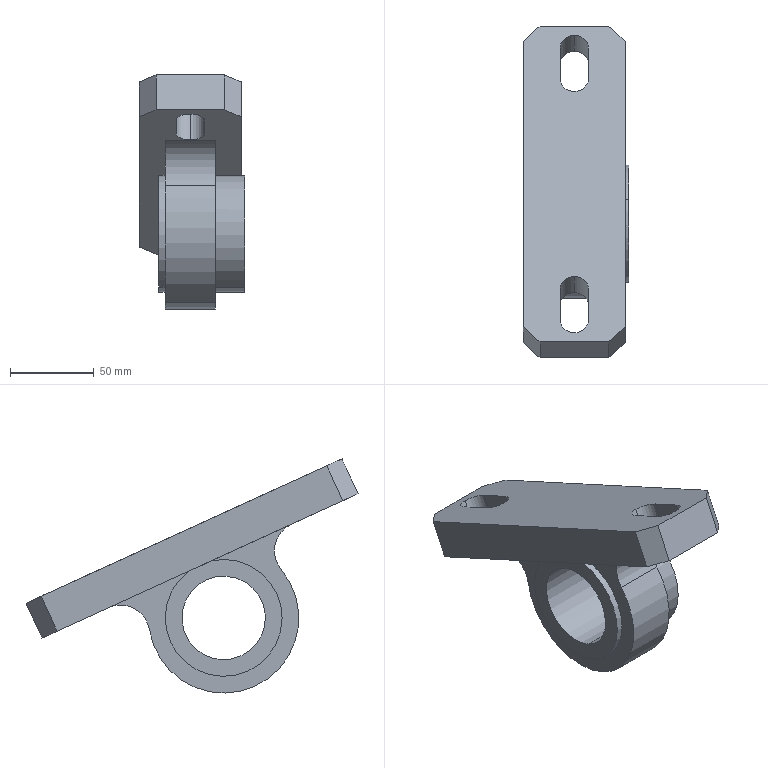Component | SolidWorks | Z90510-1 | 1 solid | 34 faces | box 63.1 x 198.79 x 140.2 mm | volume 431152 mm3 | plane 18 | cylinder 16 | commonest cylinder face diameters 17 x6 70 x4 90 x2 50 x2 35 x2
STEP:
#1=COLOUR_RGB('',0.7922,0.8196,0.9333);
#2=FILL_AREA_STYLE_COLOUR('',#1);
#3=FILL_AREA_STYLE('',(#2));
#4=SURFACE_STYLE_FILL_AREA(#3);
#5=SURFACE_SIDE_STYLE('',(#4));
#6=SURFACE_STYLE_USAGE(.BOTH.,#5);
#7=PRESENTATION_STYLE_ASSIGNMENT((#6));
#8=CARTESIAN_POINT('',(27.492,0.6244,-1.612));
#9=VERTEX_POINT('',#8);
#10=CARTESIAN_POINT('',(27.492,3.109,-0.2777));
#11=VERTEX_POINT('',#10);
#12=CARTESIAN_POINT('',(27.492,1.36,0.));
#13=DIRECTION('',(1.,0.,0.));
#14=DIRECTION('',(0.,0.4149,0.9099));
#15=AXIS2_PLACEMENT_3D('',#12,#13,#14);
#16=CIRCLE('',#15,1.772);
#17=EDGE_CURVE('',#9,#11,#16,.T.);
#18=ORIENTED_EDGE('',*,*,#17,.F.);
#19=CARTESIAN_POINT('',(26.311,0.6244,-1.612));
#20=VERTEX_POINT('',#19);
#21=CARTESIAN_POINT('',(27.374,0.6244,-1.612));
#22=DIRECTION('',(-1.,0.,0.));
#23=VECTOR('',#22,39.37);
#24=LINE('',#21,#23);
#25=EDGE_CURVE('',#9,#20,#24,.T.);
#26=ORIENTED_EDGE('',*,*,#25,.T.);
#27=CARTESIAN_POINT('',(26.311,3.109,-0.2777));
#28=VERTEX_POINT('',#27);
#29=CARTESIAN_POINT('',(26.311,1.36,0.));
#30=DIRECTION('',(1.,0.,0.));
#31=DIRECTION('',(0.,0.4149,0.9099));
#32=AXIS2_PLACEMENT_3D('',#29,#30,#31);
#33=CIRCLE('',#32,1.772);
#34=EDGE_CURVE('',#20,#28,#33,.T.);
#35=ORIENTED_EDGE('',*,*,#34,.T.);
#36=CARTESIAN_POINT('',(27.492,3.109,-0.2777));
#37=DIRECTION('',(-1.,0.,0.));
#38=VECTOR('',#37,39.37);
#39=LINE('',#36,#38);
#40=EDGE_CURVE('',#11,#28,#39,.T.);
#41=ORIENTED_EDGE('',*,*,#40,.F.);
#42=EDGE_LOOP('',(#18,#26,#35,#41));
#43=FACE_OUTER_BOUND('',#42,.T.);
#44=CARTESIAN_POINT('',(27.374,1.36,0.));
#45=DIRECTION('',(-1.,0.,0.));
#46=DIRECTION('',(0.,-0.4149,-0.9099));
#47=AXIS2_PLACEMENT_3D('',#44,#45,#46);
#48=CYLINDRICAL_SURFACE('',#47,1.772);
#49=ADVANCED_FACE('',(#43),#48,.T.);
#50=CARTESIAN_POINT('',(26.902,5.804,0.4481));
#51=VERTEX_POINT('',#50);
#52=CARTESIAN_POINT('',(27.236,5.5,0.587));
#53=VERTEX_POINT('',#52);
#54=CARTESIAN_POINT('',(26.902,5.5,0.587));
#55=DIRECTION('',(0.,-0.4149,-0.9099));
#56=DIRECTION('',(0.,-0.9099,0.4149));
#57=AXIS2_PLACEMENT_3D('',#54,#55,#56);
#58=CIRCLE('',#57,0.3346);
#59=EDGE_CURVE('',#51,#53,#58,.T.);
#60=ORIENTED_EDGE('',*,*,#59,.F.);
#61=CARTESIAN_POINT('',(26.902,5.429,-0.3758));
#62=VERTEX_POINT('',#61);
#63=CARTESIAN_POINT('',(26.902,5.804,0.4481));
#64=DIRECTION('',(0.,-0.4149,-0.9099));
#65=VECTOR('',#64,39.37);
#66=LINE('',#63,#65);
#67=EDGE_CURVE('',#51,#62,#66,.T.);
#68=ORIENTED_EDGE('',*,*,#67,.T.);
#69=CARTESIAN_POINT('',(27.236,5.124,-0.2369));
#70=VERTEX_POINT('',#69);
#71=CARTESIAN_POINT('',(26.902,5.124,-0.2369));
#72=DIRECTION('',(0.,-0.4149,-0.9099));
#73=DIRECTION('',(0.,-0.9099,0.4149));
#74=AXIS2_PLACEMENT_3D('',#71,#72,#73);
#75=CIRCLE('',#74,0.3346);
#76=EDGE_CURVE('',#62,#70,#75,.T.);
#77=ORIENTED_EDGE('',*,*,#76,.T.);
#78=CARTESIAN_POINT('',(27.236,5.5,0.587));
#79=DIRECTION('',(0.,-0.4149,-0.9099));
#80=VECTOR('',#79,39.37);
#81=LINE('',#78,#80);
#82=EDGE_CURVE('',#53,#70,#81,.T.);
#83=ORIENTED_EDGE('',*,*,#82,.F.);
#84=EDGE_LOOP('',(#60,#68,#77,#83));
#85=FACE_OUTER_BOUND('',#84,.T.);
#86=CARTESIAN_POINT('',(26.902,5.5,0.587));
#87=DIRECTION('',(0.,-0.4149,-0.9099));
#88=DIRECTION('',(0.,0.9099,-0.4149));
#89=AXIS2_PLACEMENT_3D('',#86,#87,#88);
#90=CYLINDRICAL_SURFACE('',#89,0.3346);
#91=ADVANCED_FACE('',(#85),#90,.F.);
#92=CARTESIAN_POINT('',(26.902,0.1088,3.045));
#93=VERTEX_POINT('',#92);
#94=CARTESIAN_POINT('',(27.236,-0.1957,3.184));
#95=VERTEX_POINT('',#94);
#96=CARTESIAN_POINT('',(26.902,-0.1957,3.184));
#97=DIRECTION('',(0.,-0.4149,-0.9099));
#98=DIRECTION('',(0.,0.9099,-0.4149));
#99=AXIS2_PLACEMENT_3D('',#96,#97,#98);
#100=CIRCLE('',#99,0.3346);
#101=EDGE_CURVE('',#93,#95,#100,.T.);
#102=ORIENTED_EDGE('',*,*,#101,.F.);
#103=CARTESIAN_POINT('',(26.902,-0.2669,2.222));
#104=VERTEX_POINT('',#103);
#105=CARTESIAN_POINT('',(26.902,0.1088,3.045));
#106=DIRECTION('',(0.,-0.4149,-0.9099));
#107=VECTOR('',#106,39.37);
#108=LINE('',#105,#107);
#109=EDGE_CURVE('',#93,#104,#108,.T.);
#110=ORIENTED_EDGE('',*,*,#109,.T.);
#111=CARTESIAN_POINT('',(27.236,-0.5714,2.36));
#112=VERTEX_POINT('',#111);
#113=CARTESIAN_POINT('',(26.902,-0.5714,2.36));
#114=DIRECTION('',(0.,-0.4149,-0.9099));
#115=DIRECTION('',(0.,0.9099,-0.4149));
#116=AXIS2_PLACEMENT_3D('',#113,#114,#115);
#117=CIRCLE('',#116,0.3346);
#118=EDGE_CURVE('',#104,#112,#117,.T.);
#119=ORIENTED_EDGE('',*,*,#118,.T.);
#120=CARTESIAN_POINT('',(27.236,-0.1957,3.184));
#121=DIRECTION('',(0.,-0.4149,-0.9099));
#122=VECTOR('',#121,39.37);
#123=LINE('',#120,#122);
#124=EDGE_CURVE('',#95,#112,#123,.T.);
#125=ORIENTED_EDGE('',*,*,#124,.F.);
#126=EDGE_LOOP('',(#102,#110,#119,#125));
#127=FACE_OUTER_BOUND('',#126,.T.);
#128=CARTESIAN_POINT('',(26.902,-0.1957,3.184));
#129=DIRECTION('',(0.,-0.4149,-0.9099));
#130=DIRECTION('',(0.,0.9099,-0.4149));
#131=AXIS2_PLACEMENT_3D('',#128,#129,#130);
#132=CYLINDRICAL_SURFACE('',#131,0.3346);
#133=ADVANCED_FACE('',(#127),#132,.F.);
#134=CARTESIAN_POINT('',(28.185,0.9511,-0.8955));
#135=VERTEX_POINT('',#134);
#136=CARTESIAN_POINT('',(28.185,1.768,0.8955));
#137=VERTEX_POINT('',#136);
#138=CARTESIAN_POINT('',(28.185,1.36,0.));
#139=DIRECTION('',(1.,0.,0.));
#140=DIRECTION('',(0.,0.4149,0.9099));
#141=AXIS2_PLACEMENT_3D('',#138,#139,#140);
#142=CIRCLE('',#141,0.9843);
#143=EDGE_CURVE('',#135,#137,#142,.T.);
#144=ORIENTED_EDGE('',*,*,#143,.T.);
#145=CARTESIAN_POINT('',(26.154,1.768,0.8955));
#146=VERTEX_POINT('',#145);
#147=CARTESIAN_POINT('',(28.185,1.768,0.8955));
#148=DIRECTION('',(-1.,0.,0.));
#149=VECTOR('',#148,39.37);
#150=LINE('',#147,#149);
#151=EDGE_CURVE('',#137,#146,#150,.T.);
#152=ORIENTED_EDGE('',*,*,#151,.T.);
#153=CARTESIAN_POINT('',(26.154,0.9511,-0.8955));
#154=VERTEX_POINT('',#153);
#155=CARTESIAN_POINT('',(26.154,1.36,0.));
#156=DIRECTION('',(1.,0.,0.));
#157=DIRECTION('',(0.,0.4149,0.9099));
#158=AXIS2_PLACEMENT_3D('',#155,#156,#157);
#159=CIRCLE('',#158,0.9843);
#160=EDGE_CURVE('',#154,#146,#159,.T.);
#161=ORIENTED_EDGE('',*,*,#160,.F.);
#162=CARTESIAN_POINT('',(28.185,0.9511,-0.8955));
#163=DIRECTION('',(-1.,0.,0.));
#164=VECTOR('',#163,39.37);
#165=LINE('',#162,#164);
#166=EDGE_CURVE('',#135,#154,#165,.T.);
#167=ORIENTED_EDGE('',*,*,#166,.F.);
#168=EDGE_LOOP('',(#144,#152,#161,#167));
#169=FACE_OUTER_BOUND('',#168,.T.);
#170=CARTESIAN_POINT('',(28.185,1.36,0.));
#171=DIRECTION('',(-1.,0.,0.));
#172=DIRECTION('',(0.,-0.4149,-0.9099));
#173=AXIS2_PLACEMENT_3D('',#170,#171,#172);
#174=CYLINDRICAL_SURFACE('',#173,0.9843);
#175=ADVANCED_FACE('',(#169),#174,.F.);
#176=CARTESIAN_POINT('',(28.185,1.931,1.254));
#177=VERTEX_POINT('',#176);
#178=CARTESIAN_POINT('',(28.185,0.7878,-1.254));
#179=VERTEX_POINT('',#178);
#180=CARTESIAN_POINT('',(28.185,1.36,0.));
#181=DIRECTION('',(1.,0.,0.));
#182=DIRECTION('',(0.,0.4149,0.9099));
#183=AXIS2_PLACEMENT_3D('',#180,#181,#182);
#184=CIRCLE('',#183,1.378);
#185=EDGE_CURVE('',#177,#179,#184,.T.);
#186=ORIENTED_EDGE('',*,*,#185,.F.);
#187=CARTESIAN_POINT('',(28.102,1.931,1.254));
#188=VERTEX_POINT('',#187);
#189=CARTESIAN_POINT('',(28.185,1.931,1.254));
#190=DIRECTION('',(-1.,0.,0.));
#191=VECTOR('',#190,39.37);
#192=LINE('',#189,#191);
#193=EDGE_CURVE('',#177,#188,#192,.T.);
#194=ORIENTED_EDGE('',*,*,#193,.T.);
#195=CARTESIAN_POINT('',(28.102,1.652,1.347));
#196=VERTEX_POINT('',#195);
#197=CARTESIAN_POINT('',(28.102,1.36,0.));
#198=DIRECTION('',(1.,0.,0.));
#199=DIRECTION('',(0.,0.4149,0.9099));
#200=AXIS2_PLACEMENT_3D('',#197,#198,#199);
#201=CIRCLE('',#200,1.378);
#202=EDGE_CURVE('',#188,#196,#201,.T.);
#203=ORIENTED_EDGE('',*,*,#202,.T.);
#204=CARTESIAN_POINT('',(27.492,1.652,1.347));
#205=VERTEX_POINT('',#204);
#206=CARTESIAN_POINT('',(28.185,1.652,1.347));
#207=DIRECTION('',(1.,0.,0.));
#208=VECTOR('',#207,39.37);
#209=LINE('',#206,#208);
#210=EDGE_CURVE('',#205,#196,#209,.T.);
#211=ORIENTED_EDGE('',*,*,#210,.F.);
#212=CARTESIAN_POINT('',(27.492,0.7878,-1.254));
#213=VERTEX_POINT('',#212);
#214=CARTESIAN_POINT('',(27.492,1.36,0.));
#215=DIRECTION('',(1.,0.,0.));
#216=DIRECTION('',(0.,0.4149,0.9099));
#217=AXIS2_PLACEMENT_3D('',#214,#215,#216);
#218=CIRCLE('',#217,1.378);
#219=EDGE_CURVE('',#205,#213,#218,.T.);
#220=ORIENTED_EDGE('',*,*,#219,.T.);
#221=CARTESIAN_POINT('',(28.185,0.7878,-1.254));
#222=DIRECTION('',(-1.,0.,0.));
#223=VECTOR('',#222,39.37);
#224=LINE('',#221,#223);
#225=EDGE_CURVE('',#179,#213,#224,.T.);
#226=ORIENTED_EDGE('',*,*,#225,.F.);
#227=EDGE_LOOP('',(#186,#194,#203,#211,#220,#226));
#228=FACE_OUTER_BOUND('',#227,.T.);
#229=CARTESIAN_POINT('',(28.185,1.36,0.));
#230=DIRECTION('',(-1.,0.,0.));
#231=DIRECTION('',(0.,-0.4149,-0.9099));
#232=AXIS2_PLACEMENT_3D('',#229,#230,#231);
#233=CYLINDRICAL_SURFACE('',#232,1.378);
#234=ADVANCED_FACE('',(#228),#233,.T.);
#235=CARTESIAN_POINT('',(26.311,0.7878,-1.254));
#236=VERTEX_POINT('',#235);
#237=CARTESIAN_POINT('',(26.311,2.185,1.104));
#238=VERTEX_POINT('',#237);
#239=CARTESIAN_POINT('',(26.311,1.36,0.));
#240=DIRECTION('',(1.,0.,0.));
#241=DIRECTION('',(0.,0.4149,0.9099));
#242=AXIS2_PLACEMENT_3D('',#239,#240,#241);
#243=CIRCLE('',#242,1.378);
#244=EDGE_CURVE('',#236,#238,#243,.T.);
#245=ORIENTED_EDGE('',*,*,#244,.F.);
#246=CARTESIAN_POINT('',(26.154,0.7878,-1.254));
#247=VERTEX_POINT('',#246);
#248=CARTESIAN_POINT('',(28.185,0.7878,-1.254));
#249=DIRECTION('',(-1.,0.,0.));
#250=VECTOR('',#249,39.37);
#251=LINE('',#248,#250);
#252=EDGE_CURVE('',#236,#247,#251,.T.);
#253=ORIENTED_EDGE('',*,*,#252,.T.);
#254=CARTESIAN_POINT('',(26.154,2.185,1.104));
#255=VERTEX_POINT('',#254);
#256=CARTESIAN_POINT('',(26.154,1.36,0.));
#257=DIRECTION('',(1.,0.,0.));
#258=DIRECTION('',(0.,0.4149,0.9099));
#259=AXIS2_PLACEMENT_3D('',#256,#257,#258);
#260=CIRCLE('',#259,1.378);
#261=EDGE_CURVE('',#247,#255,#260,.T.);
#262=ORIENTED_EDGE('',*,*,#261,.T.);
#263=CARTESIAN_POINT('',(28.185,2.185,1.104));
#264=DIRECTION('',(-1.,0.,0.));
#265=VECTOR('',#264,39.37);
#266=LINE('',#263,#265);
#267=EDGE_CURVE('',#238,#255,#266,.T.);
#268=ORIENTED_EDGE('',*,*,#267,.F.);
#269=EDGE_LOOP('',(#245,#253,#262,#268));
#270=FACE_OUTER_BOUND('',#269,.T.);
#271=CARTESIAN_POINT('',(28.185,1.36,0.));
#272=DIRECTION('',(-1.,0.,0.));
#273=DIRECTION('',(0.,-0.4149,-0.9099));
#274=AXIS2_PLACEMENT_3D('',#271,#272,#273);
#275=CYLINDRICAL_SURFACE('',#274,1.378);
#276=ADVANCED_FACE('',(#270),#275,.T.);
#277=ORIENTED_EDGE('',*,*,#252,.F.);
#278=CARTESIAN_POINT('',(26.311,1.652,1.347));
#279=VERTEX_POINT('',#278);
#280=CARTESIAN_POINT('',(26.311,1.36,0.));
#281=DIRECTION('',(1.,0.,0.));
#282=DIRECTION('',(0.,0.4149,0.9099));
#283=AXIS2_PLACEMENT_3D('',#280,#281,#282);
#284=CIRCLE('',#283,1.378);
#285=EDGE_CURVE('',#279,#236,#284,.T.);
#286=ORIENTED_EDGE('',*,*,#285,.F.);
#287=CARTESIAN_POINT('',(26.154,1.652,1.347));
#288=VERTEX_POINT('',#287);
#289=CARTESIAN_POINT('',(28.185,1.652,1.347));
#290=DIRECTION('',(1.,0.,0.));
#291=VECTOR('',#290,39.37);
#292=LINE('',#289,#291);
#293=EDGE_CURVE('',#288,#279,#292,.T.);
#294=ORIENTED_EDGE('',*,*,#293,.F.);
#295=CARTESIAN_POINT('',(26.154,1.36,0.));
#296=DIRECTION('',(1.,0.,0.));
#297=DIRECTION('',(0.,0.4149,0.9099));
#298=AXIS2_PLACEMENT_3D('',#295,#296,#297);
#299=CIRCLE('',#298,1.378);
#300=EDGE_CURVE('',#288,#247,#299,.T.);
#301=ORIENTED_EDGE('',*,*,#300,.T.);
#302=EDGE_LOOP('',(#277,#286,#294,#301));
#303=FACE_OUTER_BOUND('',#302,.T.);
#304=CARTESIAN_POINT('',(28.185,1.36,0.));
#305=DIRECTION('',(-1.,0.,0.));
#306=DIRECTION('',(0.,-0.4149,-0.9099));
#307=AXIS2_PLACEMENT_3D('',#304,#305,#306);
#308=CYLINDRICAL_SURFACE('',#307,1.378);
#309=ADVANCED_FACE('',(#303),#308,.T.);
#310=ORIENTED_EDGE('',*,*,#193,.F.);
#311=CARTESIAN_POINT('',(28.185,1.36,0.));
#312=DIRECTION('',(1.,0.,0.));
#313=DIRECTION('',(0.,0.4149,0.9099));
#314=AXIS2_PLACEMENT_3D('',#311,#312,#313);
#315=CIRCLE('',#314,1.378);
#316=EDGE_CURVE('',#179,#177,#315,.T.);
#317=ORIENTED_EDGE('',*,*,#316,.F.);
#318=ORIENTED_EDGE('',*,*,#225,.T.);
#319=CARTESIAN_POINT('',(27.492,2.185,1.104));
#320=VERTEX_POINT('',#319);
#321=CARTESIAN_POINT('',(27.492,1.36,0.));
#322=DIRECTION('',(1.,0.,0.));
#323=DIRECTION('',(0.,0.4149,0.9099));
#324=AXIS2_PLACEMENT_3D('',#321,#322,#323);
#325=CIRCLE('',#324,1.378);
#326=EDGE_CURVE('',#213,#320,#325,.T.);
#327=ORIENTED_EDGE('',*,*,#326,.T.);
#328=CARTESIAN_POINT('',(28.102,2.185,1.104));
#329=VERTEX_POINT('',#328);
#330=CARTESIAN_POINT('',(28.185,2.185,1.104));
#331=DIRECTION('',(-1.,0.,0.));
#332=VECTOR('',#331,39.37);
#333=LINE('',#330,#332);
#334=EDGE_CURVE('',#329,#320,#333,.T.);
#335=ORIENTED_EDGE('',*,*,#334,.F.);
#336=CARTESIAN_POINT('',(28.102,1.36,0.));
#337=DIRECTION('',(1.,0.,0.));
#338=DIRECTION('',(0.,0.4149,0.9099));
#339=AXIS2_PLACEMENT_3D('',#336,#337,#338);
#340=CIRCLE('',#339,1.378);
#341=EDGE_CURVE('',#329,#188,#340,.T.);
#342=ORIENTED_EDGE('',*,*,#341,.T.);
#343=EDGE_LOOP('',(#310,#317,#318,#327,#335,#342));
#344=FACE_OUTER_BOUND('',#343,.T.);
#345=CARTESIAN_POINT('',(28.185,1.36,0.));
#346=DIRECTION('',(-1.,0.,0.));
#347=DIRECTION('',(0.,-0.4149,-0.9099));
#348=AXIS2_PLACEMENT_3D('',#345,#346,#347);
#349=CYLINDRICAL_SURFACE('',#348,1.378);
#350=ADVANCED_FACE('',(#344),#349,.T.);
#351=ORIENTED_EDGE('',*,*,#160,.T.);
#352=CARTESIAN_POINT('',(26.154,1.36,0.));
#353=DIRECTION('',(1.,0.,0.));
#354=DIRECTION('',(0.,0.4149,0.9099));
#355=AXIS2_PLACEMENT_3D('',#352,#353,#354);
#356=CIRCLE('',#355,0.9843);
#357=EDGE_CURVE('',#146,#154,#356,.T.);
#358=ORIENTED_EDGE('',*,*,#357,.T.);
#359=EDGE_LOOP('',(#351,#358));
#360=FACE_BOUND('',#359,.T.);
#361=CARTESIAN_POINT('',(26.154,1.918,1.225));
#362=DIRECTION('',(0.,-0.9099,0.4149));
#363=VECTOR('',#362,39.37);
#364=LINE('',#361,#363);
#365=EDGE_CURVE('',#255,#288,#364,.T.);
#366=ORIENTED_EDGE('',*,*,#365,.F.);
#367=ORIENTED_EDGE('',*,*,#261,.F.);
#368=ORIENTED_EDGE('',*,*,#300,.F.);
#369=EDGE_LOOP('',(#366,#367,#368));
#370=FACE_OUTER_BOUND('',#369,.T.);
#371=CARTESIAN_POINT('',(26.154,1.36,0.));
#372=DIRECTION('',(1.,0.,0.));
#373=DIRECTION('',(0.,0.4149,0.9099));
#374=AXIS2_PLACEMENT_3D('',#371,#372,#373);
#375=PLANE('',#374);
#376=ADVANCED_FACE('',(#360,#370),#375,.F.);
#377=ORIENTED_EDGE('',*,*,#316,.T.);
#378=ORIENTED_EDGE('',*,*,#185,.T.);
#379=EDGE_LOOP('',(#377,#378));
#380=FACE_OUTER_BOUND('',#379,.T.);
#381=ORIENTED_EDGE('',*,*,#143,.F.);
#382=CARTESIAN_POINT('',(28.185,1.36,0.));
#383=DIRECTION('',(1.,0.,0.));
#384=DIRECTION('',(0.,0.4149,0.9099));
#385=AXIS2_PLACEMENT_3D('',#382,#383,#384);
#386=CIRCLE('',#385,0.9843);
#387=EDGE_CURVE('',#137,#135,#386,.T.);
#388=ORIENTED_EDGE('',*,*,#387,.F.);
#389=EDGE_LOOP('',(#381,#388));
#390=FACE_BOUND('',#389,.T.);
#391=CARTESIAN_POINT('',(28.185,1.36,0.));
#392=DIRECTION('',(1.,0.,0.));
#393=DIRECTION('',(0.,0.4149,0.9099));
#394=AXIS2_PLACEMENT_3D('',#391,#392,#393);
#395=PLANE('',#394);
#396=ADVANCED_FACE('',(#380,#390),#395,.T.);
#397=ORIENTED_EDGE('',*,*,#151,.F.);
#398=ORIENTED_EDGE('',*,*,#387,.T.);
#399=ORIENTED_EDGE('',*,*,#166,.T.);
#400=ORIENTED_EDGE('',*,*,#357,.F.);
#401=EDGE_LOOP('',(#397,#398,#399,#400));
#402=FACE_OUTER_BOUND('',#401,.T.);
#403=CARTESIAN_POINT('',(28.185,1.36,0.));
#404=DIRECTION('',(-1.,0.,0.));
#405=DIRECTION('',(0.,-0.4149,-0.9099));
#406=AXIS2_PLACEMENT_3D('',#403,#404,#405);
#407=CYLINDRICAL_SURFACE('',#406,0.9843);
#408=ADVANCED_FACE('',(#402),#407,.F.);
#409=CARTESIAN_POINT('',(28.102,5.285,-0.3104));
#410=VERTEX_POINT('',#409);
#411=CARTESIAN_POINT('',(28.102,5.644,-0.4738));
#412=DIRECTION('',(0.,0.9099,-0.4149));
#413=VECTOR('',#412,39.37);
#414=LINE('',#411,#413);
#415=EDGE_CURVE('',#329,#410,#414,.T.);
#416=ORIENTED_EDGE('',*,*,#415,.T.);
#417=CARTESIAN_POINT('',(28.102,5.661,0.5134));
#418=VERTEX_POINT('',#417);
#419=CARTESIAN_POINT('',(28.102,5.661,0.5134));
#420=DIRECTION('',(0.,0.4149,0.9099));
#421=VECTOR('',#420,39.37);
#422=LINE('',#419,#421);
#423=EDGE_CURVE('',#410,#418,#422,.T.);
#424=ORIENTED_EDGE('',*,*,#423,.T.);
#425=CARTESIAN_POINT('',(28.102,-1.073,3.585));
#426=VERTEX_POINT('',#425);
#427=CARTESIAN_POINT('',(28.102,6.019,0.3501));
#428=DIRECTION('',(0.,-0.9099,0.4149));
#429=VECTOR('',#428,39.37);
#430=LINE('',#427,#429);
#431=EDGE_CURVE('',#418,#426,#430,.T.);
#432=ORIENTED_EDGE('',*,*,#431,.T.);
#433=CARTESIAN_POINT('',(28.102,-1.449,2.761));
#434=VERTEX_POINT('',#433);
#435=CARTESIAN_POINT('',(28.102,-1.449,2.761));
#436=DIRECTION('',(0.,-0.4149,-0.9099));
#437=VECTOR('',#436,39.37);
#438=LINE('',#435,#437);
#439=EDGE_CURVE('',#426,#434,#438,.T.);
#440=ORIENTED_EDGE('',*,*,#439,.T.);
#441=CARTESIAN_POINT('',(28.102,5.644,-0.4738));
#442=DIRECTION('',(0.,0.9099,-0.4149));
#443=VECTOR('',#442,39.37);
#444=LINE('',#441,#443);
#445=EDGE_CURVE('',#434,#196,#444,.T.);
#446=ORIENTED_EDGE('',*,*,#445,.T.);
#447=ORIENTED_EDGE('',*,*,#202,.F.);
#448=ORIENTED_EDGE('',*,*,#341,.F.);
#449=EDGE_LOOP('',(#416,#424,#432,#440,#446,#447,#448));
#450=FACE_OUTER_BOUND('',#449,.T.);
#451=CARTESIAN_POINT('',(28.102,1.36,0.));
#452=DIRECTION('',(1.,0.,0.));
#453=DIRECTION('',(0.,0.4149,0.9099));
#454=AXIS2_PLACEMENT_3D('',#451,#452,#453);
#455=PLANE('',#454);
#456=ADVANCED_FACE('',(#450),#455,.T.);
#457=CARTESIAN_POINT('',(25.701,-1.449,2.761));
#458=VERTEX_POINT('',#457);
#459=CARTESIAN_POINT('',(25.701,5.285,-0.3104));
#460=VERTEX_POINT('',#459);
#461=CARTESIAN_POINT('',(25.701,5.644,-0.4738));
#462=DIRECTION('',(0.,0.9099,-0.4149));
#463=VECTOR('',#462,39.37);
#464=LINE('',#461,#463);
#465=EDGE_CURVE('',#458,#460,#464,.T.);
#466=ORIENTED_EDGE('',*,*,#465,.T.);
#467=CARTESIAN_POINT('',(26.095,5.644,-0.4738));
#468=VERTEX_POINT('',#467);
#469=CARTESIAN_POINT('',(26.095,5.644,-0.4738));
#470=DIRECTION('',(0.7071,0.6434,-0.2934));
#471=VECTOR('',#470,39.37);
#472=LINE('',#469,#471);
#473=EDGE_CURVE('',#460,#468,#472,.T.);
#474=ORIENTED_EDGE('',*,*,#473,.T.);
#475=CARTESIAN_POINT('',(27.709,5.644,-0.4738));
#476=VERTEX_POINT('',#475);
#477=CARTESIAN_POINT('',(28.102,5.644,-0.4738));
#478=DIRECTION('',(-1.,0.,0.));
#479=VECTOR('',#478,39.37);
#480=LINE('',#477,#479);
#481=EDGE_CURVE('',#476,#468,#480,.T.);
#482=ORIENTED_EDGE('',*,*,#481,.F.);
#483=CARTESIAN_POINT('',(28.102,5.285,-0.3104));
#484=DIRECTION('',(0.7071,-0.6434,0.2934));
#485=VECTOR('',#484,39.37);
#486=LINE('',#483,#485);
#487=EDGE_CURVE('',#476,#410,#486,.T.);
#488=ORIENTED_EDGE('',*,*,#487,.T.);
#489=ORIENTED_EDGE('',*,*,#415,.F.);
#490=ORIENTED_EDGE('',*,*,#334,.T.);
#491=CARTESIAN_POINT('',(27.492,4.076,0.2412));
#492=VERTEX_POINT('',#491);
#493=CARTESIAN_POINT('',(27.492,-0.2392,2.209));
#494=DIRECTION('',(0.,-0.9099,0.4149));
#495=VECTOR('',#494,39.37);
#496=LINE('',#493,#495);
#497=EDGE_CURVE('',#492,#320,#496,.T.);
#498=ORIENTED_EDGE('',*,*,#497,.F.);
#499=CARTESIAN_POINT('',(26.311,4.076,0.2412));
#500=VERTEX_POINT('',#499);
#501=CARTESIAN_POINT('',(27.492,4.076,0.2412));
#502=DIRECTION('',(-1.,0.,0.));
#503=VECTOR('',#502,39.37);
#504=LINE('',#501,#503);
#505=EDGE_CURVE('',#492,#500,#504,.T.);
#506=ORIENTED_EDGE('',*,*,#505,.T.);
#507=CARTESIAN_POINT('',(26.311,-0.2392,2.209));
#508=DIRECTION('',(0.,-0.9099,0.4149));
#509=VECTOR('',#508,39.37);
#510=LINE('',#507,#509);
#511=EDGE_CURVE('',#500,#238,#510,.T.);
#512=ORIENTED_EDGE('',*,*,#511,.T.);
#513=ORIENTED_EDGE('',*,*,#267,.T.);
#514=ORIENTED_EDGE('',*,*,#365,.T.);
#515=ORIENTED_EDGE('',*,*,#293,.T.);
#516=CARTESIAN_POINT('',(26.311,-0.2392,2.209));
#517=VERTEX_POINT('',#516);
#518=CARTESIAN_POINT('',(26.311,5.644,-0.4738));
#519=DIRECTION('',(0.,0.9099,-0.4149));
#520=VECTOR('',#519,39.37);
#521=LINE('',#518,#520);
#522=EDGE_CURVE('',#517,#279,#521,.T.);
#523=ORIENTED_EDGE('',*,*,#522,.F.);
#524=CARTESIAN_POINT('',(27.492,-0.2392,2.209));
#525=VERTEX_POINT('',#524);
#526=CARTESIAN_POINT('',(27.492,-0.2392,2.209));
#527=DIRECTION('',(-1.,0.,0.));
#528=VECTOR('',#527,39.37);
#529=LINE('',#526,#528);
#530=EDGE_CURVE('',#525,#517,#529,.T.);
#531=ORIENTED_EDGE('',*,*,#530,.F.);
#532=CARTESIAN_POINT('',(27.492,5.644,-0.4738));
#533=DIRECTION('',(0.,0.9099,-0.4149));
#534=VECTOR('',#533,39.37);
#535=LINE('',#532,#534);
#536=EDGE_CURVE('',#525,#205,#535,.T.);
#537=ORIENTED_EDGE('',*,*,#536,.T.);
#538=ORIENTED_EDGE('',*,*,#210,.T.);
#539=ORIENTED_EDGE('',*,*,#445,.F.);
#540=CARTESIAN_POINT('',(27.709,-1.807,2.924));
#541=VERTEX_POINT('',#540);
#542=CARTESIAN_POINT('',(28.102,-1.449,2.761));
#543=DIRECTION('',(-0.7071,-0.6434,0.2934));
#544=VECTOR('',#543,39.37);
#545=LINE('',#542,#544);
#546=EDGE_CURVE('',#434,#541,#545,.T.);
#547=ORIENTED_EDGE('',*,*,#546,.T.);
#548=CARTESIAN_POINT('',(26.095,-1.807,2.924));
#549=VERTEX_POINT('',#548);
#550=CARTESIAN_POINT('',(28.102,-1.807,2.924));
#551=DIRECTION('',(-1.,0.,0.));
#552=VECTOR('',#551,39.37);
#553=LINE('',#550,#552);
#554=EDGE_CURVE('',#541,#549,#553,.T.);
#555=ORIENTED_EDGE('',*,*,#554,.T.);
#556=CARTESIAN_POINT('',(26.095,-1.807,2.924));
#557=DIRECTION('',(-0.7071,0.6434,-0.2934));
#558=VECTOR('',#557,39.37);
#559=LINE('',#556,#558);
#560=EDGE_CURVE('',#549,#458,#559,.T.);
#561=ORIENTED_EDGE('',*,*,#560,.T.);
#562=EDGE_LOOP('',(#466,#474,#482,#488,#489,#490,#498,#506,#512,#513,#514,#515,#523,#531,#537,#538,#539,#547,#555,#561));
#563=FACE_OUTER_BOUND('',#562,.T.);
#564=CARTESIAN_POINT('',(26.567,4.408,0.08977));
#565=VERTEX_POINT('',#564);
#566=CARTESIAN_POINT('',(26.567,5.124,-0.2369));
#567=VERTEX_POINT('',#566);
#568=CARTESIAN_POINT('',(26.567,5.124,-0.2369));
#569=DIRECTION('',(-0.,0.9099,-0.4149));
#570=VECTOR('',#569,39.37);
#571=LINE('',#568,#570);
#572=EDGE_CURVE('',#565,#567,#571,.T.);
#573=ORIENTED_EDGE('',*,*,#572,.F.);
#574=CARTESIAN_POINT('',(27.236,4.408,0.08977));
#575=VERTEX_POINT('',#574);
#576=CARTESIAN_POINT('',(26.902,4.408,0.08977));
#577=DIRECTION('',(0.,-0.4149,-0.9099));
#578=DIRECTION('',(0.,-0.9099,0.4149));
#579=AXIS2_PLACEMENT_3D('',#576,#577,#578);
#580=CIRCLE('',#579,0.3346);
#581=EDGE_CURVE('',#575,#565,#580,.T.);
#582=ORIENTED_EDGE('',*,*,#581,.F.);
#583=CARTESIAN_POINT('',(27.236,5.124,-0.2369));
#584=DIRECTION('',(-0.,-0.9099,0.4149));
#585=VECTOR('',#584,39.37);
#586=LINE('',#583,#585);
#587=EDGE_CURVE('',#70,#575,#586,.T.);
#588=ORIENTED_EDGE('',*,*,#587,.F.);
#589=ORIENTED_EDGE('',*,*,#76,.F.);
#590=CARTESIAN_POINT('',(26.902,5.124,-0.2369));
#591=DIRECTION('',(0.,-0.4149,-0.9099));
#592=DIRECTION('',(0.,-0.9099,0.4149));
#593=AXIS2_PLACEMENT_3D('',#590,#591,#592);
#594=CIRCLE('',#593,0.3346);
#595=EDGE_CURVE('',#567,#62,#594,.T.);
#596=ORIENTED_EDGE('',*,*,#595,.F.);
#597=EDGE_LOOP('',(#573,#582,#588,#589,#596));
#598=FACE_BOUND('',#597,.T.);
#599=CARTESIAN_POINT('',(26.567,-1.288,2.687));
#600=VERTEX_POINT('',#599);
#601=CARTESIAN_POINT('',(26.567,-0.5714,2.36));
#602=VERTEX_POINT('',#601);
#603=CARTESIAN_POINT('',(26.567,-1.288,2.687));
#604=DIRECTION('',(0.,0.9099,-0.4149));
#605=VECTOR('',#604,39.37);
#606=LINE('',#603,#605);
#607=EDGE_CURVE('',#600,#602,#606,.T.);
#608=ORIENTED_EDGE('',*,*,#607,.F.);
#609=CARTESIAN_POINT('',(27.236,-1.288,2.687));
#610=VERTEX_POINT('',#609);
#611=CARTESIAN_POINT('',(26.902,-1.288,2.687));
#612=DIRECTION('',(0.,-0.4149,-0.9099));
#613=DIRECTION('',(0.,0.9099,-0.4149));
#614=AXIS2_PLACEMENT_3D('',#611,#612,#613);
#615=CIRCLE('',#614,0.3346);
#616=EDGE_CURVE('',#610,#600,#615,.T.);
#617=ORIENTED_EDGE('',*,*,#616,.F.);
#618=CARTESIAN_POINT('',(27.236,-1.288,2.687));
#619=DIRECTION('',(0.,-0.9099,0.4149));
#620=VECTOR('',#619,39.37);
#621=LINE('',#618,#620);
#622=EDGE_CURVE('',#112,#610,#621,.T.);
#623=ORIENTED_EDGE('',*,*,#622,.F.);
#624=ORIENTED_EDGE('',*,*,#118,.F.);
#625=CARTESIAN_POINT('',(26.902,-0.5714,2.36));
#626=DIRECTION('',(0.,-0.4149,-0.9099));
#627=DIRECTION('',(0.,0.9099,-0.4149));
#628=AXIS2_PLACEMENT_3D('',#625,#626,#627);
#629=CIRCLE('',#628,0.3346);
#630=EDGE_CURVE('',#602,#104,#629,.T.);
#631=ORIENTED_EDGE('',*,*,#630,.F.);
#632=EDGE_LOOP('',(#608,#617,#623,#624,#631));
#633=FACE_BOUND('',#632,.T.);
#634=CARTESIAN_POINT('',(28.102,5.644,-0.4738));
#635=DIRECTION('',(0.,0.4149,0.9099));
#636=DIRECTION('',(0.,-0.9099,0.4149));
#637=AXIS2_PLACEMENT_3D('',#634,#635,#636);
#638=PLANE('',#637);
#639=ADVANCED_FACE('',(#563,#598,#633),#638,.F.);
#640=ORIENTED_EDGE('',*,*,#481,.T.);
#641=CARTESIAN_POINT('',(26.095,6.019,0.3501));
#642=VERTEX_POINT('',#641);
#643=CARTESIAN_POINT('',(26.095,5.644,-0.4738));
#644=DIRECTION('',(0.,0.4149,0.9099));
#645=VECTOR('',#644,39.37);
#646=LINE('',#643,#645);
#647=EDGE_CURVE('',#468,#642,#646,.T.);
#648=ORIENTED_EDGE('',*,*,#647,.T.);
#649=CARTESIAN_POINT('',(27.709,6.019,0.3501));
#650=VERTEX_POINT('',#649);
#651=CARTESIAN_POINT('',(28.102,6.019,0.3501));
#652=DIRECTION('',(-1.,0.,0.));
#653=VECTOR('',#652,39.37);
#654=LINE('',#651,#653);
#655=EDGE_CURVE('',#650,#642,#654,.T.);
#656=ORIENTED_EDGE('',*,*,#655,.F.);
#657=CARTESIAN_POINT('',(27.709,5.644,-0.4738));
#658=DIRECTION('',(0.,-0.4149,-0.9099));
#659=VECTOR('',#658,39.37);
#660=LINE('',#657,#659);
#661=EDGE_CURVE('',#650,#476,#660,.T.);
#662=ORIENTED_EDGE('',*,*,#661,.T.);
#663=EDGE_LOOP('',(#640,#648,#656,#662));
#664=FACE_OUTER_BOUND('',#663,.T.);
#665=CARTESIAN_POINT('',(28.102,5.644,-0.4738));
#666=DIRECTION('',(0.,-0.9099,0.4149));
#667=DIRECTION('',(0.,-0.4149,-0.9099));
#668=AXIS2_PLACEMENT_3D('',#665,#666,#667);
#669=PLANE('',#668);
#670=ADVANCED_FACE('',(#664),#669,.F.);
#671=CARTESIAN_POINT('',(27.236,4.783,0.9137));
#672=VERTEX_POINT('',#671);
#673=CARTESIAN_POINT('',(27.236,5.5,0.587));
#674=DIRECTION('',(-0.,-0.9099,0.4149));
#675=VECTOR('',#674,39.37);
#676=LINE('',#673,#675);
#677=EDGE_CURVE('',#53,#672,#676,.T.);
#678=ORIENTED_EDGE('',*,*,#677,.T.);
#679=CARTESIAN_POINT('',(26.567,4.783,0.9137));
#680=VERTEX_POINT('',#679);
#681=CARTESIAN_POINT('',(26.902,4.783,0.9137));
#682=DIRECTION('',(0.,-0.4149,-0.9099));
#683=DIRECTION('',(0.,-0.9099,0.4149));
#684=AXIS2_PLACEMENT_3D('',#681,#682,#683);
#685=CIRCLE('',#684,0.3346);
#686=EDGE_CURVE('',#672,#680,#685,.T.);
#687=ORIENTED_EDGE('',*,*,#686,.T.);
#688=CARTESIAN_POINT('',(26.567,5.5,0.587));
#689=VERTEX_POINT('',#688);
#690=CARTESIAN_POINT('',(26.567,5.5,0.587));
#691=DIRECTION('',(-0.,0.9099,-0.4149));
#692=VECTOR('',#691,39.37);
#693=LINE('',#690,#692);
#694=EDGE_CURVE('',#680,#689,#693,.T.);
#695=ORIENTED_EDGE('',*,*,#694,.T.);
#696=CARTESIAN_POINT('',(26.902,5.5,0.587));
#697=DIRECTION('',(0.,-0.4149,-0.9099));
#698=DIRECTION('',(0.,-0.9099,0.4149));
#699=AXIS2_PLACEMENT_3D('',#696,#697,#698);
#700=CIRCLE('',#699,0.3346);
#701=EDGE_CURVE('',#689,#51,#700,.T.);
#702=ORIENTED_EDGE('',*,*,#701,.T.);
#703=ORIENTED_EDGE('',*,*,#59,.T.);
#704=EDGE_LOOP('',(#678,#687,#695,#702,#703));
#705=FACE_BOUND('',#704,.T.);
#706=CARTESIAN_POINT('',(27.236,-0.9121,3.511));
#707=VERTEX_POINT('',#706);
#708=CARTESIAN_POINT('',(27.236,-0.9121,3.511));
#709=DIRECTION('',(0.,-0.9099,0.4149));
#710=VECTOR('',#709,39.37);
#711=LINE('',#708,#710);
#712=EDGE_CURVE('',#95,#707,#711,.T.);
#713=ORIENTED_EDGE('',*,*,#712,.T.);
#714=CARTESIAN_POINT('',(26.567,-0.9121,3.511));
#715=VERTEX_POINT('',#714);
#716=CARTESIAN_POINT('',(26.902,-0.9121,3.511));
#717=DIRECTION('',(0.,-0.4149,-0.9099));
#718=DIRECTION('',(0.,0.9099,-0.4149));
#719=AXIS2_PLACEMENT_3D('',#716,#717,#718);
#720=CIRCLE('',#719,0.3346);
#721=EDGE_CURVE('',#707,#715,#720,.T.);
#722=ORIENTED_EDGE('',*,*,#721,.T.);
#723=CARTESIAN_POINT('',(26.567,-0.1957,3.184));
#724=VERTEX_POINT('',#723);
#725=CARTESIAN_POINT('',(26.567,-0.9121,3.511));
#726=DIRECTION('',(0.,0.9099,-0.4149));
#727=VECTOR('',#726,39.37);
#728=LINE('',#725,#727);
#729=EDGE_CURVE('',#715,#724,#728,.T.);
#730=ORIENTED_EDGE('',*,*,#729,.T.);
#731=CARTESIAN_POINT('',(26.902,-0.1957,3.184));
#732=DIRECTION('',(0.,-0.4149,-0.9099));
#733=DIRECTION('',(0.,0.9099,-0.4149));
#734=AXIS2_PLACEMENT_3D('',#731,#732,#733);
#735=CIRCLE('',#734,0.3346);
#736=EDGE_CURVE('',#724,#93,#735,.T.);
#737=ORIENTED_EDGE('',*,*,#736,.T.);
#738=ORIENTED_EDGE('',*,*,#101,.T.);
#739=EDGE_LOOP('',(#713,#722,#730,#737,#738));
#740=FACE_BOUND('',#739,.T.);
#741=ORIENTED_EDGE('',*,*,#655,.T.);
#742=CARTESIAN_POINT('',(25.701,5.661,0.5134));
#743=VERTEX_POINT('',#742);
#744=CARTESIAN_POINT('',(26.095,6.019,0.3501));
#745=DIRECTION('',(-0.7071,-0.6434,0.2934));
#746=VECTOR('',#745,39.37);
#747=LINE('',#744,#746);
#748=EDGE_CURVE('',#642,#743,#747,.T.);
#749=ORIENTED_EDGE('',*,*,#748,.T.);
#750=CARTESIAN_POINT('',(25.701,-1.073,3.585));
#751=VERTEX_POINT('',#750);
#752=CARTESIAN_POINT('',(25.701,6.019,0.3501));
#753=DIRECTION('',(0.,-0.9099,0.4149));
#754=VECTOR('',#753,39.37);
#755=LINE('',#752,#754);
#756=EDGE_CURVE('',#743,#751,#755,.T.);
#757=ORIENTED_EDGE('',*,*,#756,.T.);
#758=CARTESIAN_POINT('',(26.095,-1.432,3.748));
#759=VERTEX_POINT('',#758);
#760=CARTESIAN_POINT('',(26.095,-1.432,3.748));
#761=DIRECTION('',(0.7071,-0.6434,0.2934));
#762=VECTOR('',#761,39.37);
#763=LINE('',#760,#762);
#764=EDGE_CURVE('',#751,#759,#763,.T.);
#765=ORIENTED_EDGE('',*,*,#764,.T.);
#766=CARTESIAN_POINT('',(27.709,-1.432,3.748));
#767=VERTEX_POINT('',#766);
#768=CARTESIAN_POINT('',(28.102,-1.432,3.748));
#769=DIRECTION('',(-1.,0.,0.));
#770=VECTOR('',#769,39.37);
#771=LINE('',#768,#770);
#772=EDGE_CURVE('',#767,#759,#771,.T.);
#773=ORIENTED_EDGE('',*,*,#772,.F.);
#774=CARTESIAN_POINT('',(28.102,-1.073,3.585));
#775=DIRECTION('',(0.7071,0.6434,-0.2934));
#776=VECTOR('',#775,39.37);
#777=LINE('',#774,#776);
#778=EDGE_CURVE('',#767,#426,#777,.T.);
#779=ORIENTED_EDGE('',*,*,#778,.T.);
#780=ORIENTED_EDGE('',*,*,#431,.F.);
#781=CARTESIAN_POINT('',(28.102,5.661,0.5134));
#782=DIRECTION('',(-0.7071,0.6434,-0.2934));
#783=VECTOR('',#782,39.37);
#784=LINE('',#781,#783);
#785=EDGE_CURVE('',#418,#650,#784,.T.);
#786=ORIENTED_EDGE('',*,*,#785,.T.);
#787=EDGE_LOOP('',(#741,#749,#757,#765,#773,#779,#780,#786));
#788=FACE_OUTER_BOUND('',#787,.T.);
#789=CARTESIAN_POINT('',(28.102,6.019,0.3501));
#790=DIRECTION('',(0.,-0.4149,-0.9099));
#791=DIRECTION('',(0.,0.9099,-0.4149));
#792=AXIS2_PLACEMENT_3D('',#789,#790,#791);
#793=PLANE('',#792);
#794=ADVANCED_FACE('',(#705,#740,#788),#793,.F.);
#795=ORIENTED_EDGE('',*,*,#772,.T.);
#796=CARTESIAN_POINT('',(26.095,-1.807,2.924));
#797=DIRECTION('',(0.,-0.4149,-0.9099));
#798=VECTOR('',#797,39.37);
#799=LINE('',#796,#798);
#800=EDGE_CURVE('',#759,#549,#799,.T.);
#801=ORIENTED_EDGE('',*,*,#800,.T.);
#802=ORIENTED_EDGE('',*,*,#554,.F.);
#803=CARTESIAN_POINT('',(27.709,-1.432,3.748));
#804=DIRECTION('',(0.,0.4149,0.9099));
#805=VECTOR('',#804,39.37);
#806=LINE('',#803,#805);
#807=EDGE_CURVE('',#541,#767,#806,.T.);
#808=ORIENTED_EDGE('',*,*,#807,.T.);
#809=EDGE_LOOP('',(#795,#801,#802,#808));
#810=FACE_OUTER_BOUND('',#809,.T.);
#811=CARTESIAN_POINT('',(28.102,-1.807,2.924));
#812=DIRECTION('',(0.,0.9099,-0.4149));
#813=DIRECTION('',(0.,0.4149,0.9099));
#814=AXIS2_PLACEMENT_3D('',#811,#812,#813);
#815=PLANE('',#814);
#816=ADVANCED_FACE('',(#810),#815,.F.);
#817=ORIENTED_EDGE('',*,*,#756,.F.);
#818=CARTESIAN_POINT('',(25.701,4.727,-1.536));
#819=DIRECTION('',(0.,-0.4149,-0.9099));
#820=VECTOR('',#819,39.37);
#821=LINE('',#818,#820);
#822=EDGE_CURVE('',#743,#460,#821,.T.);
#823=ORIENTED_EDGE('',*,*,#822,.T.);
#824=ORIENTED_EDGE('',*,*,#465,.F.);
#825=CARTESIAN_POINT('',(25.701,-2.008,1.536));
#826=DIRECTION('',(0.,0.4149,0.9099));
#827=VECTOR('',#826,39.37);
#828=LINE('',#825,#827);
#829=EDGE_CURVE('',#458,#751,#828,.T.);
#830=ORIENTED_EDGE('',*,*,#829,.T.);
#831=EDGE_LOOP('',(#817,#823,#824,#830));
#832=FACE_OUTER_BOUND('',#831,.T.);
#833=CARTESIAN_POINT('',(25.701,1.36,0.));
#834=DIRECTION('',(1.,0.,0.));
#835=DIRECTION('',(0.,0.4149,0.9099));
#836=AXIS2_PLACEMENT_3D('',#833,#834,#835);
#837=PLANE('',#836);
#838=ADVANCED_FACE('',(#832),#837,.F.);
#839=ORIENTED_EDGE('',*,*,#616,.T.);
#840=CARTESIAN_POINT('',(26.567,-0.9121,3.511));
#841=DIRECTION('',(0.,-0.4149,-0.9099));
#842=VECTOR('',#841,39.37);
#843=LINE('',#840,#842);
#844=EDGE_CURVE('',#715,#600,#843,.T.);
#845=ORIENTED_EDGE('',*,*,#844,.F.);
#846=ORIENTED_EDGE('',*,*,#721,.F.);
#847=CARTESIAN_POINT('',(27.236,-0.9121,3.511));
#848=DIRECTION('',(0.,-0.4149,-0.9099));
#849=VECTOR('',#848,39.37);
#850=LINE('',#847,#849);
#851=EDGE_CURVE('',#707,#610,#850,.T.);
#852=ORIENTED_EDGE('',*,*,#851,.T.);
#853=EDGE_LOOP('',(#839,#845,#846,#852));
#854=FACE_OUTER_BOUND('',#853,.T.);
#855=CARTESIAN_POINT('',(26.902,-0.9121,3.511));
#856=DIRECTION('',(0.,-0.4149,-0.9099));
#857=DIRECTION('',(0.,0.9099,-0.4149));
#858=AXIS2_PLACEMENT_3D('',#855,#856,#857);
#859=CYLINDRICAL_SURFACE('',#858,0.3346);
#860=ADVANCED_FACE('',(#854),#859,.F.);
#861=ORIENTED_EDGE('',*,*,#622,.T.);
#862=ORIENTED_EDGE('',*,*,#851,.F.);
#863=ORIENTED_EDGE('',*,*,#712,.F.);
#864=ORIENTED_EDGE('',*,*,#124,.T.);
#865=EDGE_LOOP('',(#861,#862,#863,#864));
#866=FACE_OUTER_BOUND('',#865,.T.);
#867=CARTESIAN_POINT('',(27.236,-0.9121,3.511));
#868=DIRECTION('',(1.,0.,-0.));
#869=DIRECTION('',(-0.,0.9099,-0.4149));
#870=AXIS2_PLACEMENT_3D('',#867,#868,#869);
#871=PLANE('',#870);
#872=ADVANCED_FACE('',(#866),#871,.F.);
#873=ORIENTED_EDGE('',*,*,#109,.F.);
#874=ORIENTED_EDGE('',*,*,#736,.F.);
#875=CARTESIAN_POINT('',(26.567,-0.1957,3.184));
#876=DIRECTION('',(0.,-0.4149,-0.9099));
#877=VECTOR('',#876,39.37);
#878=LINE('',#875,#877);
#879=EDGE_CURVE('',#724,#602,#878,.T.);
#880=ORIENTED_EDGE('',*,*,#879,.T.);
#881=ORIENTED_EDGE('',*,*,#630,.T.);
#882=EDGE_LOOP('',(#873,#874,#880,#881));
#883=FACE_OUTER_BOUND('',#882,.T.);
#884=CARTESIAN_POINT('',(26.902,-0.1957,3.184));
#885=DIRECTION('',(0.,-0.4149,-0.9099));
#886=DIRECTION('',(0.,0.9099,-0.4149));
#887=AXIS2_PLACEMENT_3D('',#884,#885,#886);
#888=CYLINDRICAL_SURFACE('',#887,0.3346);
#889=ADVANCED_FACE('',(#883),#888,.F.);
#890=ORIENTED_EDGE('',*,*,#607,.T.);
#891=ORIENTED_EDGE('',*,*,#879,.F.);
#892=ORIENTED_EDGE('',*,*,#729,.F.);
#893=ORIENTED_EDGE('',*,*,#844,.T.);
#894=EDGE_LOOP('',(#890,#891,#892,#893));
#895=FACE_OUTER_BOUND('',#894,.T.);
#896=CARTESIAN_POINT('',(26.567,-0.9121,3.511));
#897=DIRECTION('',(-1.,0.,-0.));
#898=DIRECTION('',(-0.,-0.9099,0.4149));
#899=AXIS2_PLACEMENT_3D('',#896,#897,#898);
#900=PLANE('',#899);
#901=ADVANCED_FACE('',(#895),#900,.F.);
#902=ORIENTED_EDGE('',*,*,#581,.T.);
#903=CARTESIAN_POINT('',(26.567,4.783,0.9137));
#904=DIRECTION('',(0.,-0.4149,-0.9099));
#905=VECTOR('',#904,39.37);
#906=LINE('',#903,#905);
#907=EDGE_CURVE('',#680,#565,#906,.T.);
#908=ORIENTED_EDGE('',*,*,#907,.F.);
#909=ORIENTED_EDGE('',*,*,#686,.F.);
#910=CARTESIAN_POINT('',(27.236,4.783,0.9137));
#911=DIRECTION('',(0.,-0.4149,-0.9099));
#912=VECTOR('',#911,39.37);
#913=LINE('',#910,#912);
#914=EDGE_CURVE('',#672,#575,#913,.T.);
#915=ORIENTED_EDGE('',*,*,#914,.T.);
#916=EDGE_LOOP('',(#902,#908,#909,#915));
#917=FACE_OUTER_BOUND('',#916,.T.);
#918=CARTESIAN_POINT('',(26.902,4.783,0.9137));
#919=DIRECTION('',(0.,-0.4149,-0.9099));
#920=DIRECTION('',(0.,0.9099,-0.4149));
#921=AXIS2_PLACEMENT_3D('',#918,#919,#920);
#922=CYLINDRICAL_SURFACE('',#921,0.3346);
#923=ADVANCED_FACE('',(#917),#922,.F.);
#924=ORIENTED_EDGE('',*,*,#587,.T.);
#925=ORIENTED_EDGE('',*,*,#914,.F.);
#926=ORIENTED_EDGE('',*,*,#677,.F.);
#927=ORIENTED_EDGE('',*,*,#82,.T.);
#928=EDGE_LOOP('',(#924,#925,#926,#927));
#929=FACE_OUTER_BOUND('',#928,.T.);
#930=CARTESIAN_POINT('',(27.236,5.5,0.587));
#931=DIRECTION('',(1.,-0.,0.));
#932=DIRECTION('',(0.,0.9099,-0.4149));
#933=AXIS2_PLACEMENT_3D('',#930,#931,#932);
#934=PLANE('',#933);
#935=ADVANCED_FACE('',(#929),#934,.F.);
#936=ORIENTED_EDGE('',*,*,#67,.F.);
#937=ORIENTED_EDGE('',*,*,#701,.F.);
#938=CARTESIAN_POINT('',(26.567,5.5,0.587));
#939=DIRECTION('',(0.,-0.4149,-0.9099));
#940=VECTOR('',#939,39.37);
#941=LINE('',#938,#940);
#942=EDGE_CURVE('',#689,#567,#941,.T.);
#943=ORIENTED_EDGE('',*,*,#942,.T.);
#944=ORIENTED_EDGE('',*,*,#595,.T.);
#945=EDGE_LOOP('',(#936,#937,#943,#944));
#946=FACE_OUTER_BOUND('',#945,.T.);
#947=CARTESIAN_POINT('',(26.902,5.5,0.587));
#948=DIRECTION('',(0.,-0.4149,-0.9099));
#949=DIRECTION('',(0.,0.9099,-0.4149));
#950=AXIS2_PLACEMENT_3D('',#947,#948,#949);
#951=CYLINDRICAL_SURFACE('',#950,0.3346);
#952=ADVANCED_FACE('',(#946),#951,.F.);
#953=ORIENTED_EDGE('',*,*,#572,.T.);
#954=ORIENTED_EDGE('',*,*,#942,.F.);
#955=ORIENTED_EDGE('',*,*,#694,.F.);
#956=ORIENTED_EDGE('',*,*,#907,.T.);
#957=EDGE_LOOP('',(#953,#954,#955,#956));
#958=FACE_OUTER_BOUND('',#957,.T.);
#959=CARTESIAN_POINT('',(26.567,5.5,0.587));
#960=DIRECTION('',(-1.,-0.,0.));
#961=DIRECTION('',(0.,-0.9099,0.4149));
#962=AXIS2_PLACEMENT_3D('',#959,#960,#961);
#963=PLANE('',#962);
#964=ADVANCED_FACE('',(#958),#963,.F.);
#965=ORIENTED_EDGE('',*,*,#219,.F.);
#966=ORIENTED_EDGE('',*,*,#536,.F.);
#967=CARTESIAN_POINT('',(27.492,0.002583,1.139));
#968=VERTEX_POINT('',#967);
#969=CARTESIAN_POINT('',(27.492,-0.5251,1.582));
#970=DIRECTION('',(-1.,0.,0.));
#971=DIRECTION('',(0.,0.4149,0.9099));
#972=AXIS2_PLACEMENT_3D('',#969,#970,#971);
#973=CIRCLE('',#972,0.689);
#974=EDGE_CURVE('',#525,#968,#973,.T.);
#975=ORIENTED_EDGE('',*,*,#974,.T.);
#976=CARTESIAN_POINT('',(27.492,1.36,0.));
#977=DIRECTION('',(1.,0.,0.));
#978=DIRECTION('',(0.,0.4149,0.9099));
#979=AXIS2_PLACEMENT_3D('',#976,#977,#978);
#980=CIRCLE('',#979,1.772);
#981=EDGE_CURVE('',#968,#9,#980,.T.);
#982=ORIENTED_EDGE('',*,*,#981,.T.);
#983=ORIENTED_EDGE('',*,*,#17,.T.);
#984=CARTESIAN_POINT('',(27.492,3.79,-0.3856));
#985=DIRECTION('',(-1.,0.,0.));
#986=DIRECTION('',(0.,0.4149,0.9099));
#987=AXIS2_PLACEMENT_3D('',#984,#985,#986);
#988=CIRCLE('',#987,0.689);
#989=EDGE_CURVE('',#11,#492,#988,.T.);
#990=ORIENTED_EDGE('',*,*,#989,.T.);
#991=ORIENTED_EDGE('',*,*,#497,.T.);
#992=ORIENTED_EDGE('',*,*,#326,.F.);
#993=EDGE_LOOP('',(#965,#966,#975,#982,#983,#990,#991,#992));
#994=FACE_OUTER_BOUND('',#993,.T.);
#995=CARTESIAN_POINT('',(27.492,-0.5251,1.582));
#996=DIRECTION('',(1.,0.,0.));
#997=DIRECTION('',(0.,0.4149,0.9099));
#998=AXIS2_PLACEMENT_3D('',#995,#996,#997);
#999=PLANE('',#998);
#1000=ADVANCED_FACE('',(#994),#999,.T.);
#1001=ORIENTED_EDGE('',*,*,#522,.T.);
#1002=ORIENTED_EDGE('',*,*,#285,.T.);
#1003=ORIENTED_EDGE('',*,*,#244,.T.);
#1004=ORIENTED_EDGE('',*,*,#511,.F.);
#1005=CARTESIAN_POINT('',(26.311,3.79,-0.3856));
#1006=DIRECTION('',(-1.,0.,0.));
#1007=DIRECTION('',(0.,0.4149,0.9099));
#1008=AXIS2_PLACEMENT_3D('',#1005,#1006,#1007);
#1009=CIRCLE('',#1008,0.689);
#1010=EDGE_CURVE('',#28,#500,#1009,.T.);
#1011=ORIENTED_EDGE('',*,*,#1010,.F.);
#1012=ORIENTED_EDGE('',*,*,#34,.F.);
#1013=CARTESIAN_POINT('',(26.311,0.002583,1.139));
#1014=VERTEX_POINT('',#1013);
#1015=CARTESIAN_POINT('',(26.311,1.36,0.));
#1016=DIRECTION('',(1.,0.,0.));
#1017=DIRECTION('',(0.,0.4149,0.9099));
#1018=AXIS2_PLACEMENT_3D('',#1015,#1016,#1017);
#1019=CIRCLE('',#1018,1.772);
#1020=EDGE_CURVE('',#1014,#20,#1019,.T.);
#1021=ORIENTED_EDGE('',*,*,#1020,.F.);
#1022=CARTESIAN_POINT('',(26.311,-0.5251,1.582));
#1023=DIRECTION('',(-1.,0.,0.));
#1024=DIRECTION('',(0.,0.4149,0.9099));
#1025=AXIS2_PLACEMENT_3D('',#1022,#1023,#1024);
#1026=CIRCLE('',#1025,0.689);
#1027=EDGE_CURVE('',#517,#1014,#1026,.T.);
#1028=ORIENTED_EDGE('',*,*,#1027,.F.);
#1029=EDGE_LOOP('',(#1001,#1002,#1003,#1004,#1011,#1012,#1021,#1028));
#1030=FACE_OUTER_BOUND('',#1029,.T.);
#1031=CARTESIAN_POINT('',(26.311,-0.5251,1.582));
#1032=DIRECTION('',(1.,0.,0.));
#1033=DIRECTION('',(0.,0.4149,0.9099));
#1034=AXIS2_PLACEMENT_3D('',#1031,#1032,#1033);
#1035=PLANE('',#1034);
#1036=ADVANCED_FACE('',(#1030),#1035,.F.);
#1037=ORIENTED_EDGE('',*,*,#1027,.T.);
#1038=CARTESIAN_POINT('',(27.492,0.002583,1.139));
#1039=DIRECTION('',(-1.,0.,0.));
#1040=VECTOR('',#1039,39.37);
#1041=LINE('',#1038,#1040);
#1042=EDGE_CURVE('',#968,#1014,#1041,.T.);
#1043=ORIENTED_EDGE('',*,*,#1042,.F.);
#1044=ORIENTED_EDGE('',*,*,#974,.F.);
#1045=ORIENTED_EDGE('',*,*,#530,.T.);
#1046=EDGE_LOOP('',(#1037,#1043,#1044,#1045));
#1047=FACE_OUTER_BOUND('',#1046,.T.);
#1048=CARTESIAN_POINT('',(27.492,-0.5251,1.582));
#1049=DIRECTION('',(-1.,0.,0.));
#1050=DIRECTION('',(0.,-0.4149,-0.9099));
#1051=AXIS2_PLACEMENT_3D('',#1048,#1049,#1050);
#1052=CYLINDRICAL_SURFACE('',#1051,0.689);
#1053=ADVANCED_FACE('',(#1047),#1052,.F.);
#1054=ORIENTED_EDGE('',*,*,#1010,.T.);
#1055=ORIENTED_EDGE('',*,*,#505,.F.);
#1056=ORIENTED_EDGE('',*,*,#989,.F.);
#1057=ORIENTED_EDGE('',*,*,#40,.T.);
#1058=EDGE_LOOP('',(#1054,#1055,#1056,#1057));
#1059=FACE_OUTER_BOUND('',#1058,.T.);
#1060=CARTESIAN_POINT('',(27.492,3.79,-0.3856));
#1061=DIRECTION('',(-1.,0.,0.));
#1062=DIRECTION('',(0.,-0.4149,-0.9099));
#1063=AXIS2_PLACEMENT_3D('',#1060,#1061,#1062);
#1064=CYLINDRICAL_SURFACE('',#1063,0.689);
#1065=ADVANCED_FACE('',(#1059),#1064,.F.);
#1066=ORIENTED_EDGE('',*,*,#25,.F.);
#1067=ORIENTED_EDGE('',*,*,#981,.F.);
#1068=ORIENTED_EDGE('',*,*,#1042,.T.);
#1069=ORIENTED_EDGE('',*,*,#1020,.T.);
#1070=EDGE_LOOP('',(#1066,#1067,#1068,#1069));
#1071=FACE_OUTER_BOUND('',#1070,.T.);
#1072=CARTESIAN_POINT('',(27.374,1.36,0.));
#1073=DIRECTION('',(-1.,0.,0.));
#1074=DIRECTION('',(0.,-0.4149,-0.9099));
#1075=AXIS2_PLACEMENT_3D('',#1072,#1073,#1074);
#1076=CYLINDRICAL_SURFACE('',#1075,1.772);
#1077=ADVANCED_FACE('',(#1071),#1076,.T.);
#1078=ORIENTED_EDGE('',*,*,#473,.F.);
#1079=ORIENTED_EDGE('',*,*,#822,.F.);
#1080=ORIENTED_EDGE('',*,*,#748,.F.);
#1081=ORIENTED_EDGE('',*,*,#647,.F.);
#1082=EDGE_LOOP('',(#1078,#1079,#1080,#1081));
#1083=FACE_OUTER_BOUND('',#1082,.T.);
#1084=CARTESIAN_POINT('',(26.095,5.644,-0.4738));
#1085=DIRECTION('',(0.7071,-0.6434,0.2934));
#1086=DIRECTION('',(0.,0.4149,0.9099));
#1087=AXIS2_PLACEMENT_3D('',#1084,#1085,#1086);
#1088=PLANE('',#1087);
#1089=ADVANCED_FACE('',(#1083),#1088,.F.);
#1090=ORIENTED_EDGE('',*,*,#487,.F.);
#1091=ORIENTED_EDGE('',*,*,#661,.F.);
#1092=ORIENTED_EDGE('',*,*,#785,.F.);
#1093=ORIENTED_EDGE('',*,*,#423,.F.);
#1094=EDGE_LOOP('',(#1090,#1091,#1092,#1093));
#1095=FACE_OUTER_BOUND('',#1094,.T.);
#1096=CARTESIAN_POINT('',(28.102,4.727,-1.536));
#1097=DIRECTION('',(0.7071,0.6434,-0.2934));
#1098=DIRECTION('',(0.,-0.4149,-0.9099));
#1099=AXIS2_PLACEMENT_3D('',#1096,#1097,#1098);
#1100=PLANE('',#1099);
#1101=ADVANCED_FACE('',(#1095),#1100,.T.);
#1102=ORIENTED_EDGE('',*,*,#764,.F.);
#1103=ORIENTED_EDGE('',*,*,#829,.F.);
#1104=ORIENTED_EDGE('',*,*,#560,.F.);
#1105=ORIENTED_EDGE('',*,*,#800,.F.);
#1106=EDGE_LOOP('',(#1102,#1103,#1104,#1105));
#1107=FACE_OUTER_BOUND('',#1106,.T.);
#1108=CARTESIAN_POINT('',(26.095,-1.807,2.924));
#1109=DIRECTION('',(0.7071,0.6434,-0.2934));
#1110=DIRECTION('',(0.,-0.4149,-0.9099));
#1111=AXIS2_PLACEMENT_3D('',#1108,#1109,#1110);
#1112=PLANE('',#1111);
#1113=ADVANCED_FACE('',(#1107),#1112,.F.);
#1114=ORIENTED_EDGE('',*,*,#778,.F.);
#1115=ORIENTED_EDGE('',*,*,#807,.F.);
#1116=ORIENTED_EDGE('',*,*,#546,.F.);
#1117=ORIENTED_EDGE('',*,*,#439,.F.);
#1118=EDGE_LOOP('',(#1114,#1115,#1116,#1117));
#1119=FACE_OUTER_BOUND('',#1118,.T.);
#1120=CARTESIAN_POINT('',(28.102,-2.008,1.536));
#1121=DIRECTION('',(0.7071,-0.6434,0.2934));
#1122=DIRECTION('',(0.,0.4149,0.9099));
#1123=AXIS2_PLACEMENT_3D('',#1120,#1121,#1122);
#1124=PLANE('',#1123);
#1125=ADVANCED_FACE('',(#1119),#1124,.T.);
#1126=CLOSED_SHELL('',(#49,#91,#133,#175,#234,#276,#309,#350,#376,#396,#408,#456,#639,#670,#794,#816,#838,#860,#872,#889,#901,#923,#935,#952,#964,#1000,#1036,#1053,#1065,#1077,#1089,#1101,#1113,#1125));
#1127=MANIFOLD_SOLID_BREP('',#1126);
#1128=STYLED_ITEM('',(#7),#1127);
#1129=PRESENTATION_LAYER_ASSIGNMENT('','',(#1128));
#1130=CARTESIAN_POINT('',(0.,0.,0.));
#1131=DIRECTION('',(0.,0.,1.));
#1132=DIRECTION('',(1.,0.,0.));
#1133=AXIS2_PLACEMENT_3D('',#1130,#1131,#1132);
#1134=(LENGTH_UNIT()NAMED_UNIT(*)SI_UNIT($,.METRE.));
#1135=LENGTH_MEASURE_WITH_UNIT(LENGTH_MEASURE(0.0254),#1134);
#1136=DIMENSIONAL_EXPONENTS(1.,0.,0.,0.,0.,0.,0.);
#1137=(CONVERSION_BASED_UNIT('',#1135)LENGTH_UNIT()NAMED_UNIT(#1136));
#1138=UNCERTAINTY_MEASURE_WITH_UNIT(LENGTH_MEASURE(0.00001),#1137,'','');
#1139=(NAMED_UNIT(*)PLANE_ANGLE_UNIT()SI_UNIT($,.RADIAN.));
#1140=(NAMED_UNIT(*)SI_UNIT($,.STERADIAN.)SOLID_ANGLE_UNIT());
#1141=(GEOMETRIC_REPRESENTATION_CONTEXT(3)GLOBAL_UNCERTAINTY_ASSIGNED_CONTEXT((#1138))GLOBAL_UNIT_ASSIGNED_CONTEXT((#1137,#1139,#1140))REPRESENTATION_CONTEXT('',''));
#1142=ADVANCED_BREP_SHAPE_REPRESENTATION('',(#1127,#1133),#1141);
#1143=(LENGTH_UNIT()NAMED_UNIT(*)SI_UNIT($,.METRE.));
#1144=LENGTH_MEASURE_WITH_UNIT(LENGTH_MEASURE(0.0254),#1143);
#1145=DIMENSIONAL_EXPONENTS(1.,0.,0.,0.,0.,0.,0.);
#1146=(CONVERSION_BASED_UNIT('',#1144)LENGTH_UNIT()NAMED_UNIT(#1145));
#1147=UNCERTAINTY_MEASURE_WITH_UNIT(LENGTH_MEASURE(0.00001),#1146,'','');
#1148=(NAMED_UNIT(*)PLANE_ANGLE_UNIT()SI_UNIT($,.RADIAN.));
#1149=(NAMED_UNIT(*)SI_UNIT($,.STERADIAN.)SOLID_ANGLE_UNIT());
#1150=(GEOMETRIC_REPRESENTATION_CONTEXT(3)GLOBAL_UNCERTAINTY_ASSIGNED_CONTEXT((#1147))GLOBAL_UNIT_ASSIGNED_CONTEXT((#1146,#1148,#1149))REPRESENTATION_CONTEXT('',''));
#1151=MECHANICAL_DESIGN_GEOMETRIC_PRESENTATION_REPRESENTATION('',(#1128),#1150);